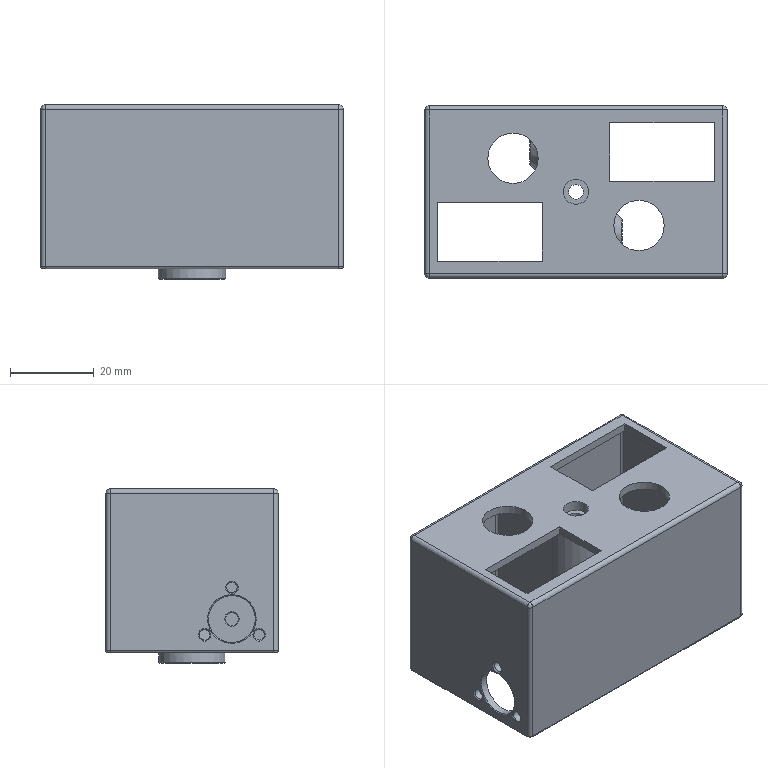Component | NX | DJZ_08_BRACKET3_TRAVEL10 | 1 solid | 148 faces | volume 25801 mm3 | cylinder 61 | plane 35 | cone 20 | sphere 14 | torus 14 | spline 4 | commonest cylinder face diameters 1 x34 2 x8 2.5 x6 12 x3 11.2 x2 12.5 x2 3.1 x2 16 x1